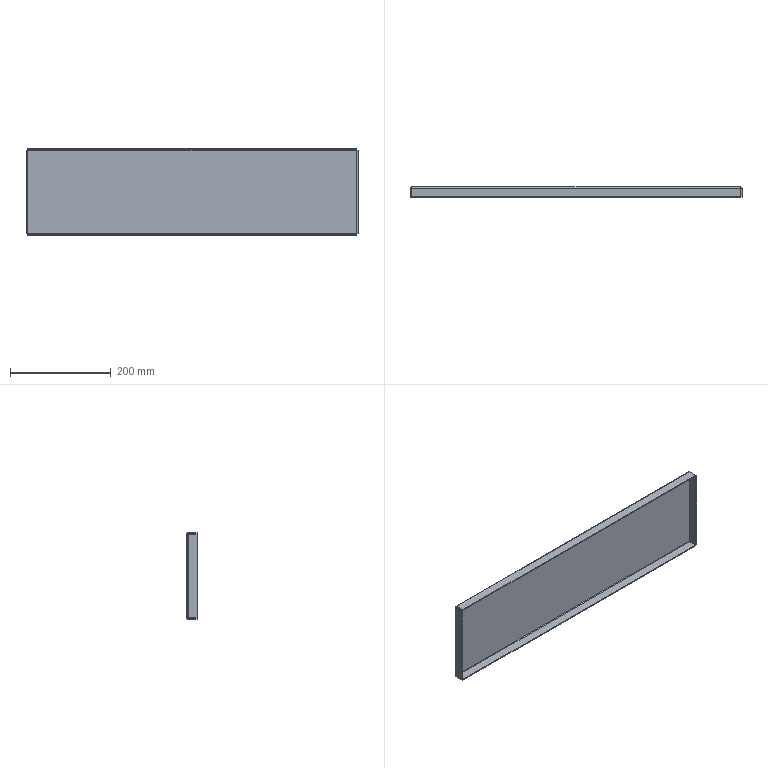Component | SolidWorks | 30-01A-1_FrontSealingPlate-1 | 1 solid | 38 faces | volume 283280 mm3 | plane 22 | spline 8 | cylinder 8 | commonest cylinder face diameters 6 x4 2 x4